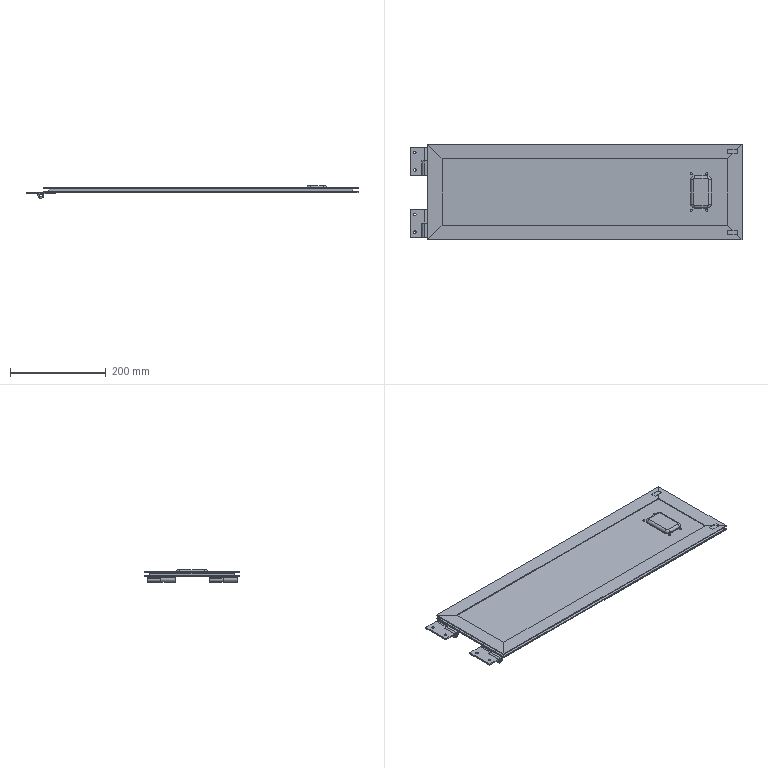Component | SolidWorks | 30-01A-1_AluminumAlloyDoorAcrylicPlate(RearDoor)-1 | 13 solids | 247 faces | volume 738629 mm3 | plane 147 | cylinder 76 | cone 16 | torus 8 | commonest cylinder face diameters 10 x16 5.5 x16 2 x16 16 x8 4.5 x8 12 x4 6 x4 4 x4